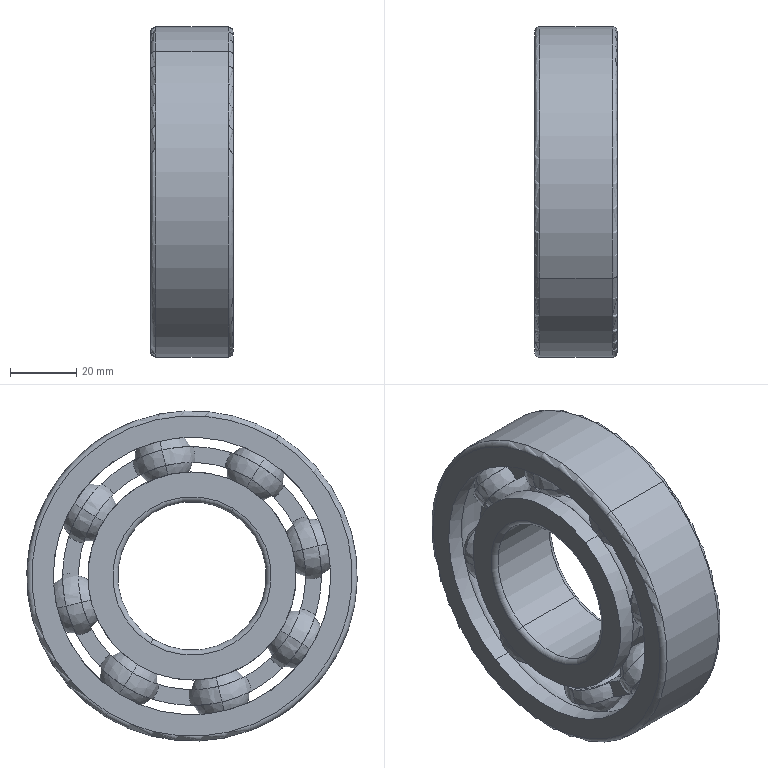Component | SolidWorks | 7DeepGrooveBallBearing276[GBT276-2013][6309]-1 | 1 solid | 132 faces | volume 105639 mm3 | sphere 64 | torus 32 | plane 20 | cylinder 16 | commonest cylinder face diameters 63 x4 84 x4 45 x2 100 x2 78.302 x2 68.698 x2 | material GCr4